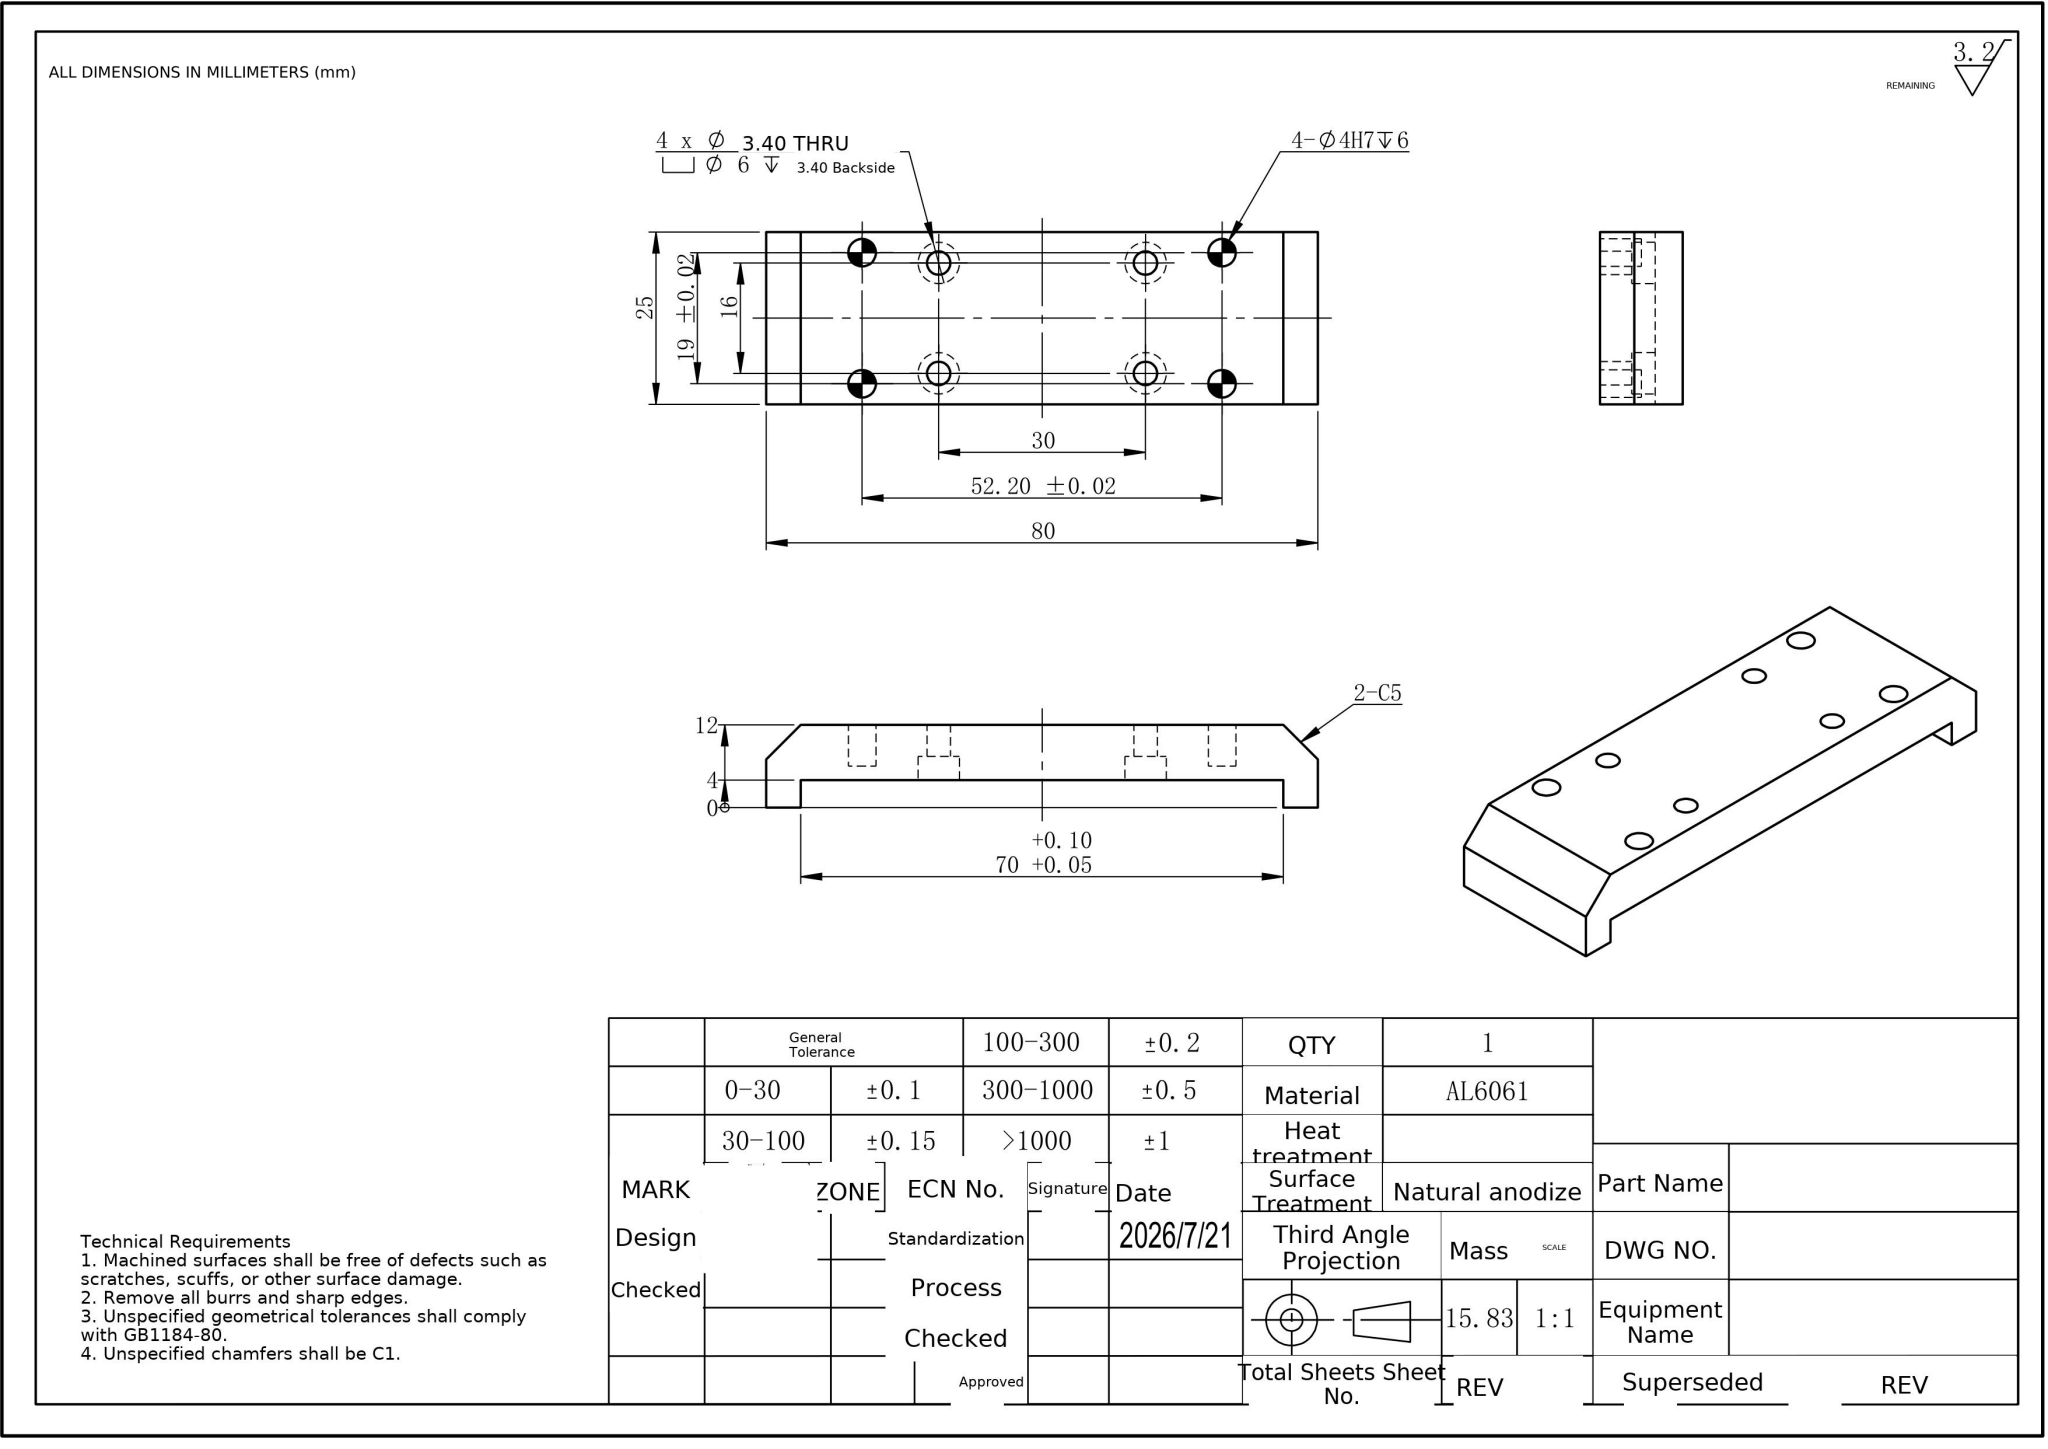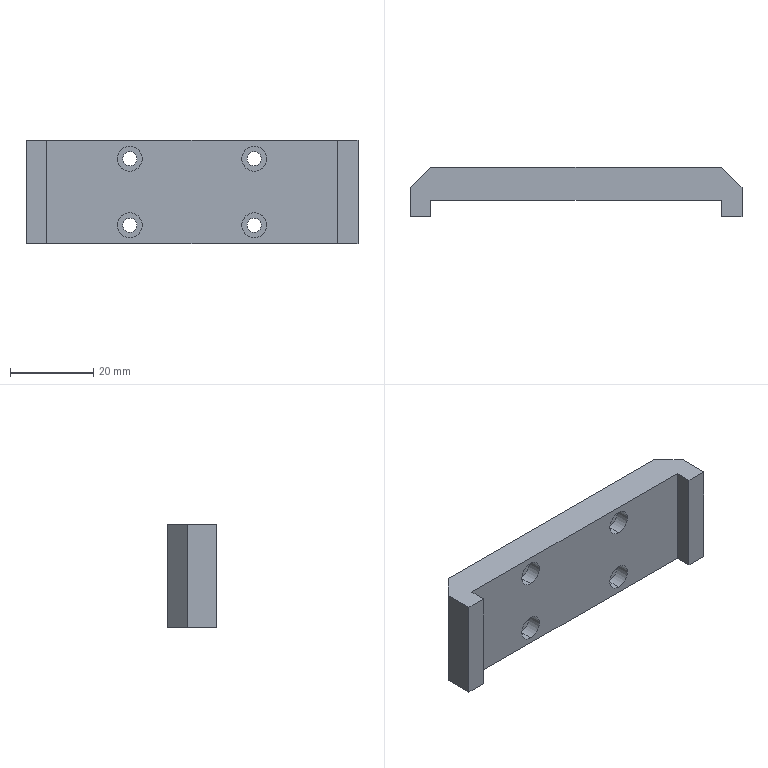Part | NX | mm | 1 solid | 44 faces | box 80 x 12 x 25 mm | volume 15522 mm3 | cylinder 24 | plane 20 | commonest cylinder face diameters 4 x8 6 x8 3.4 x8